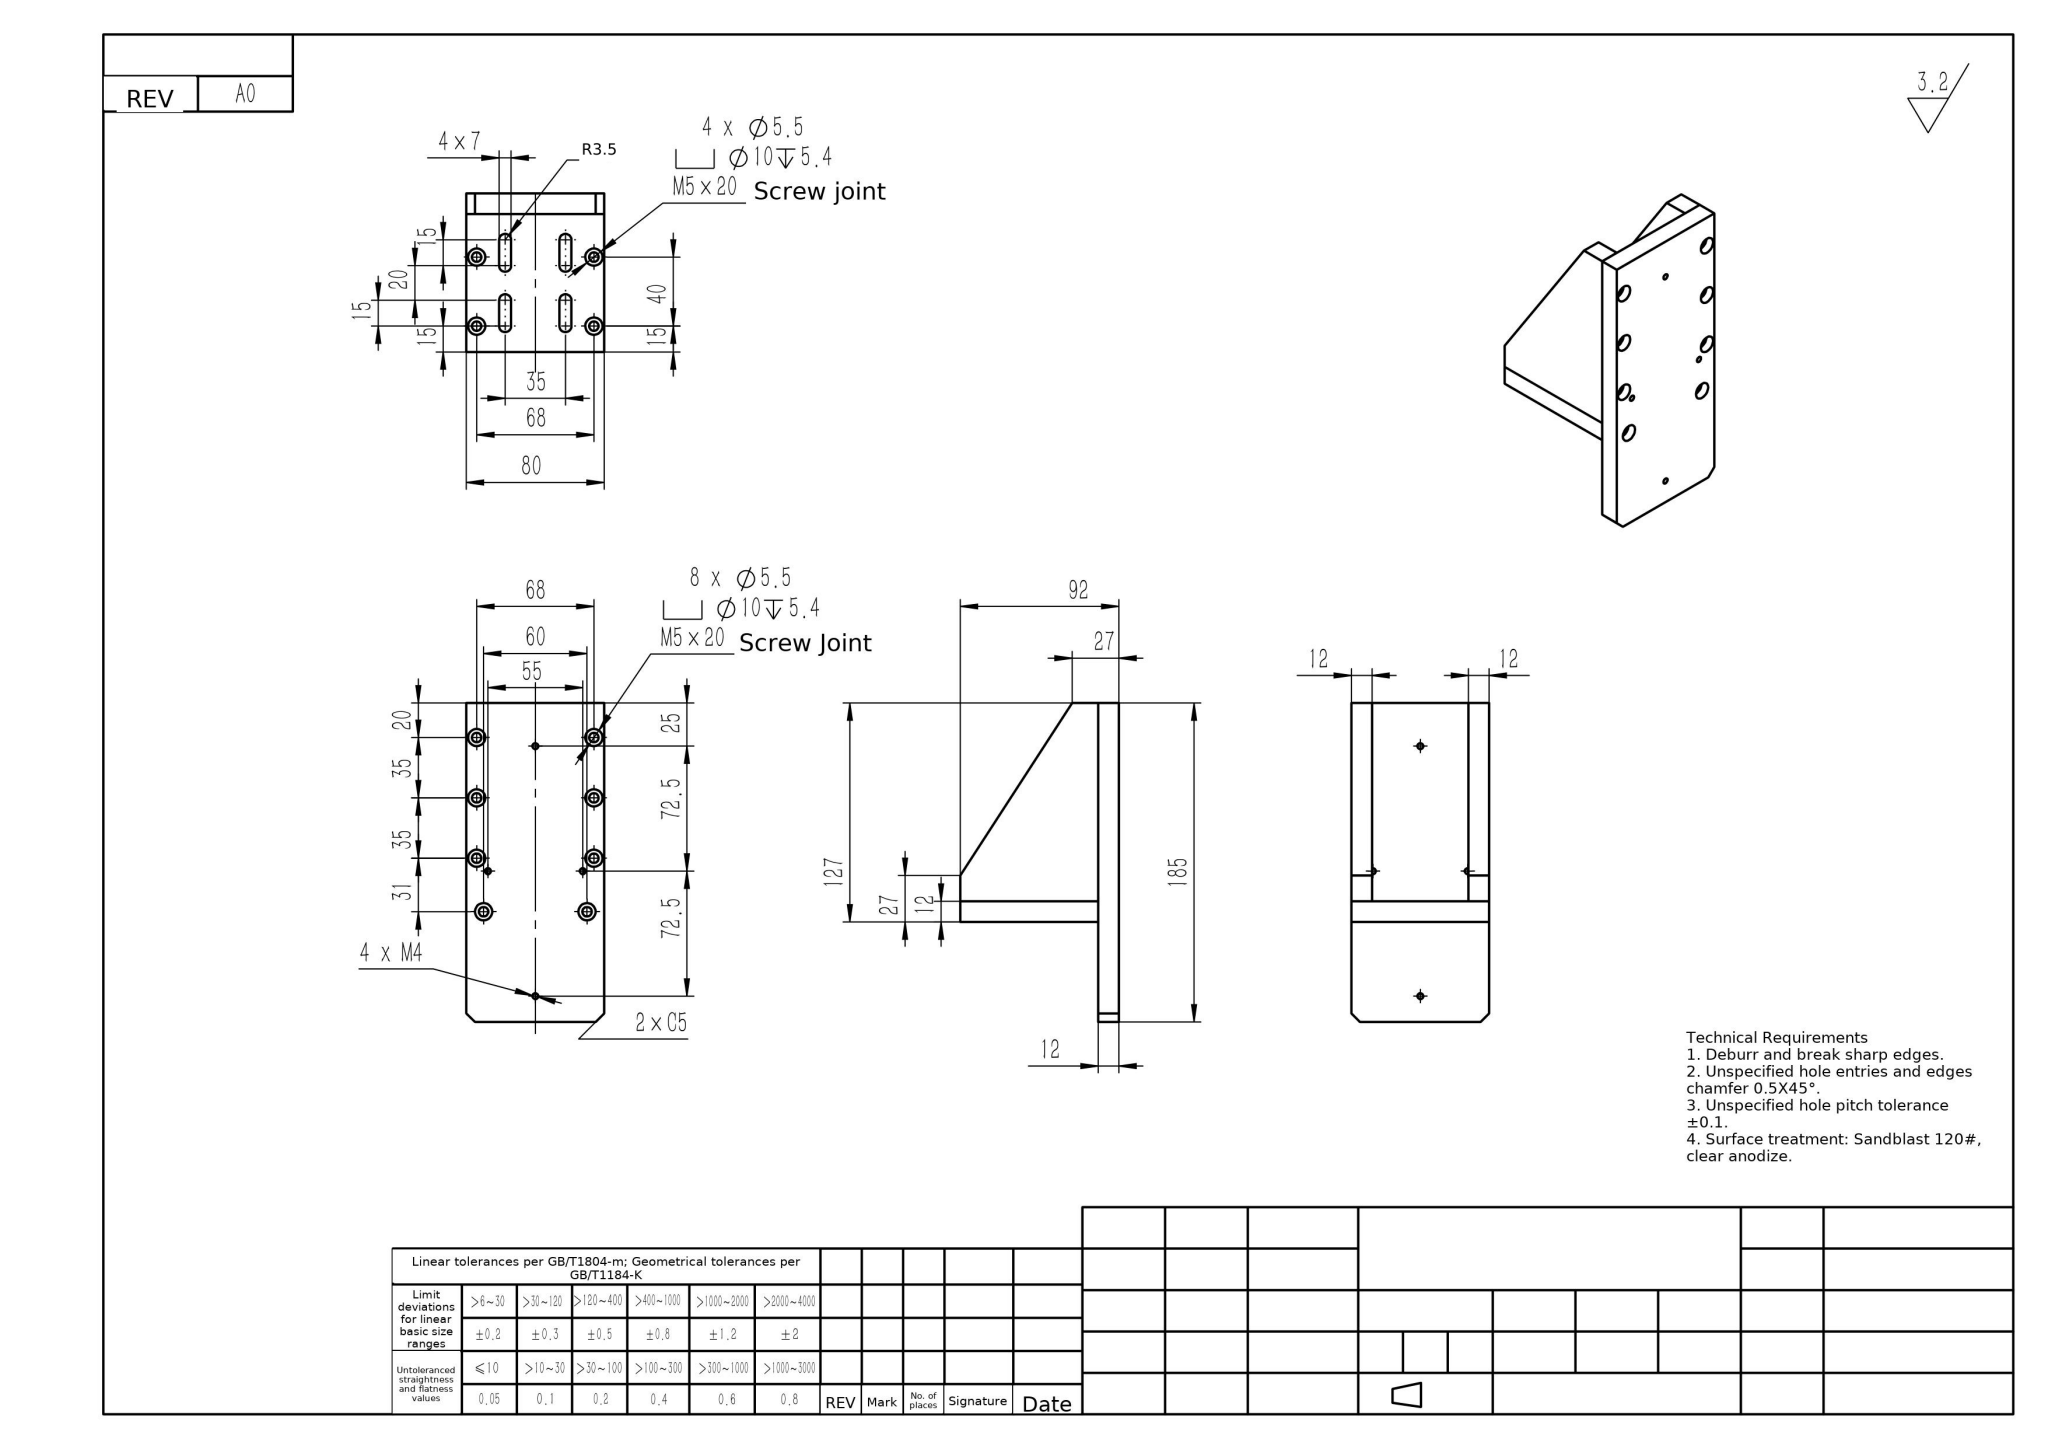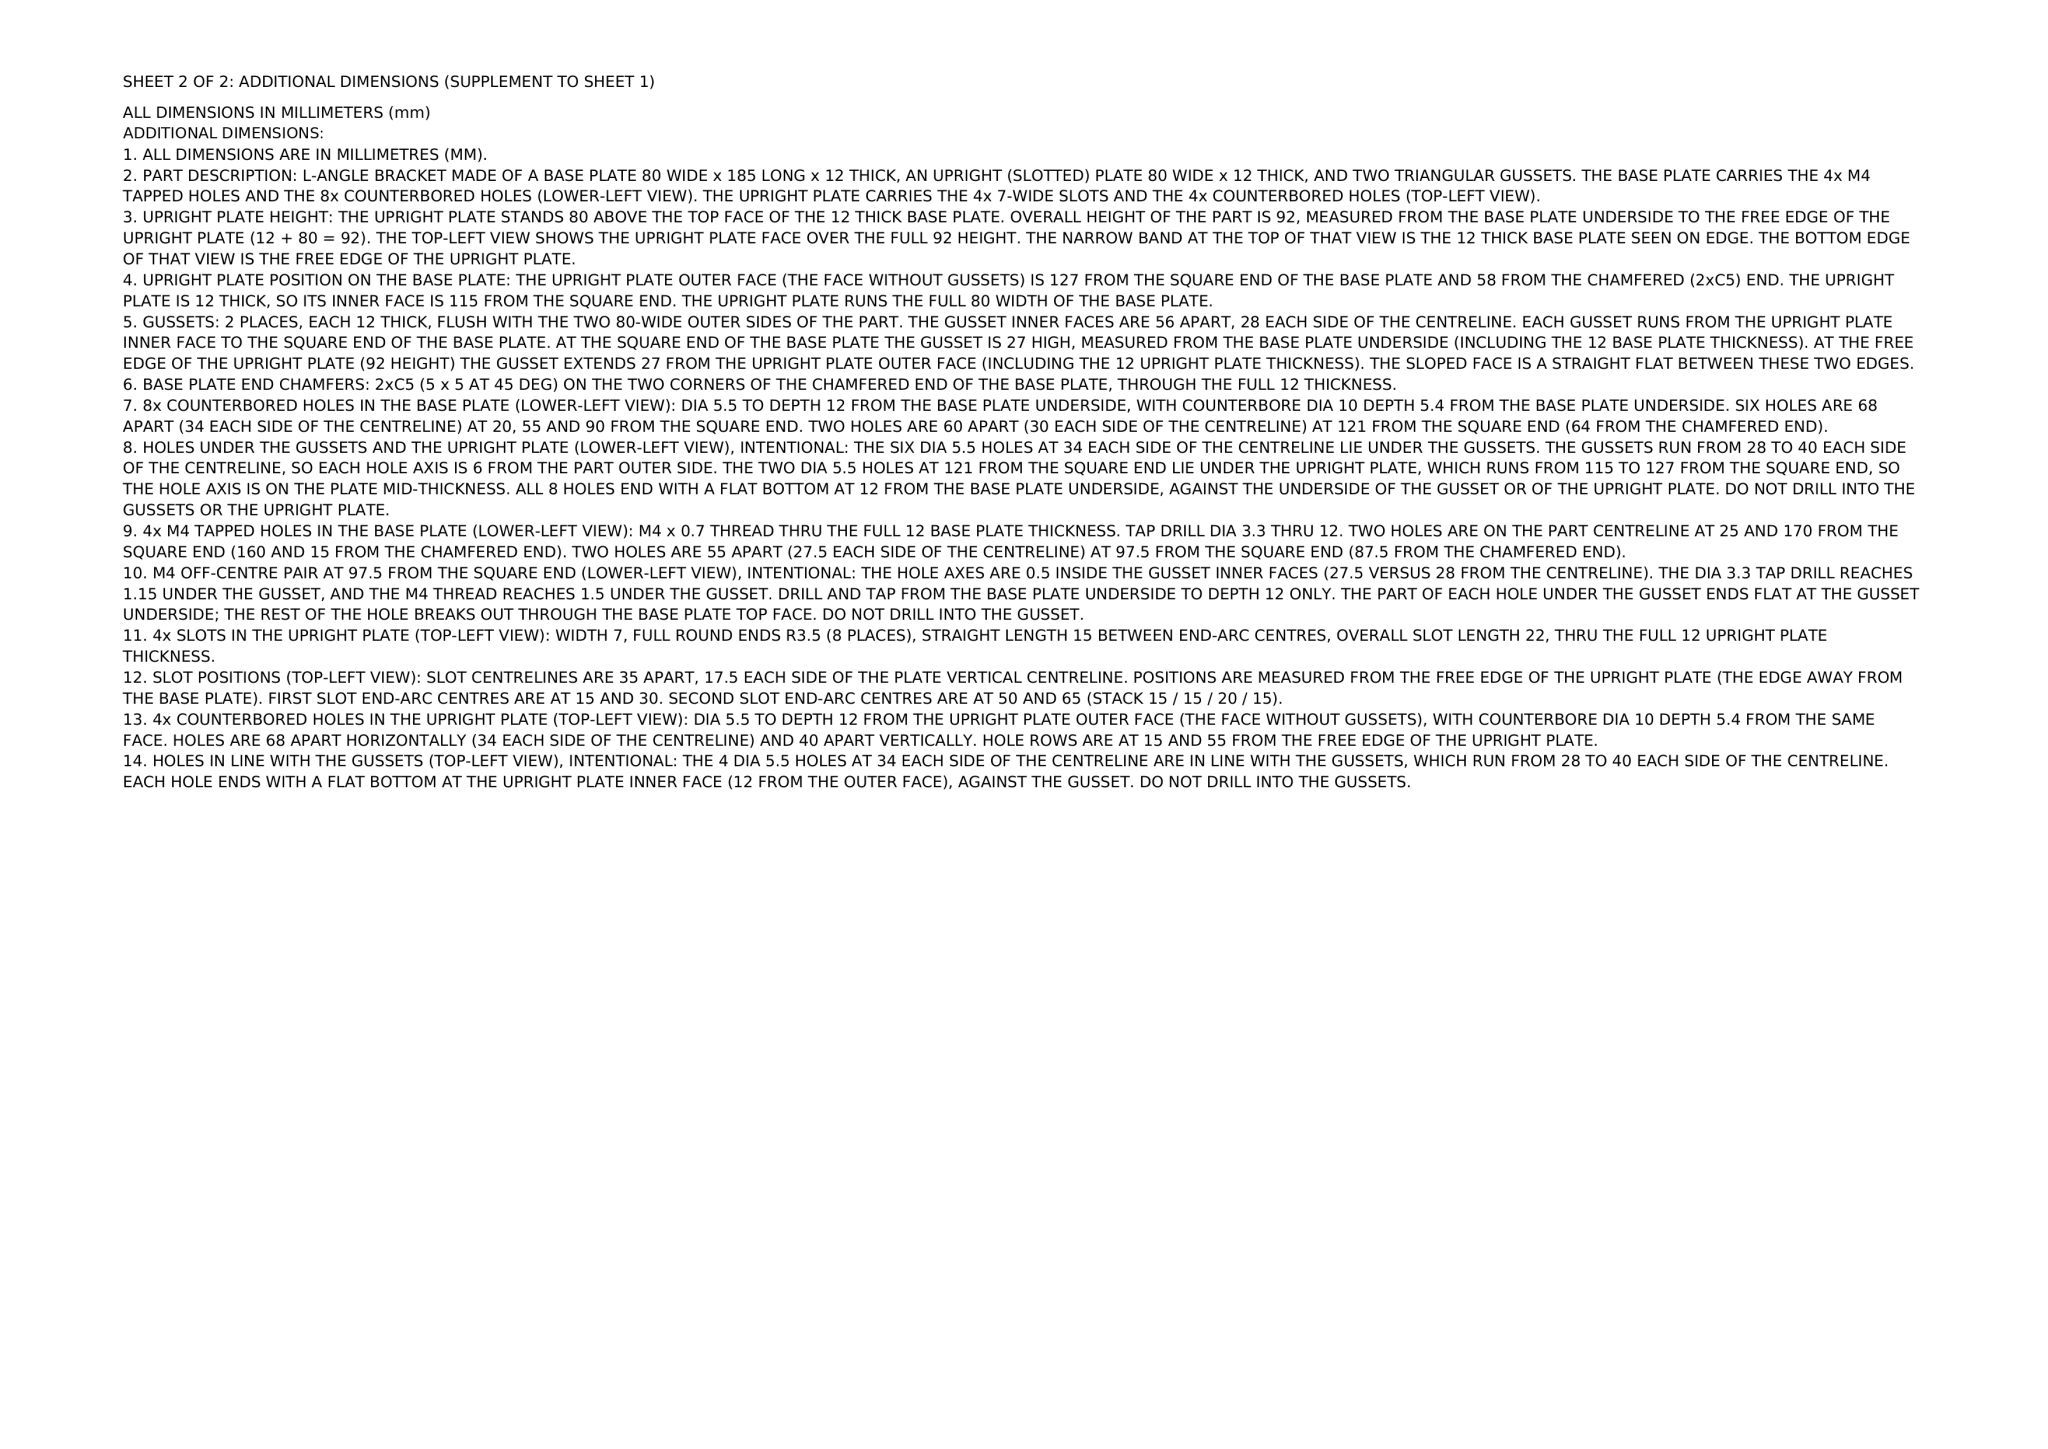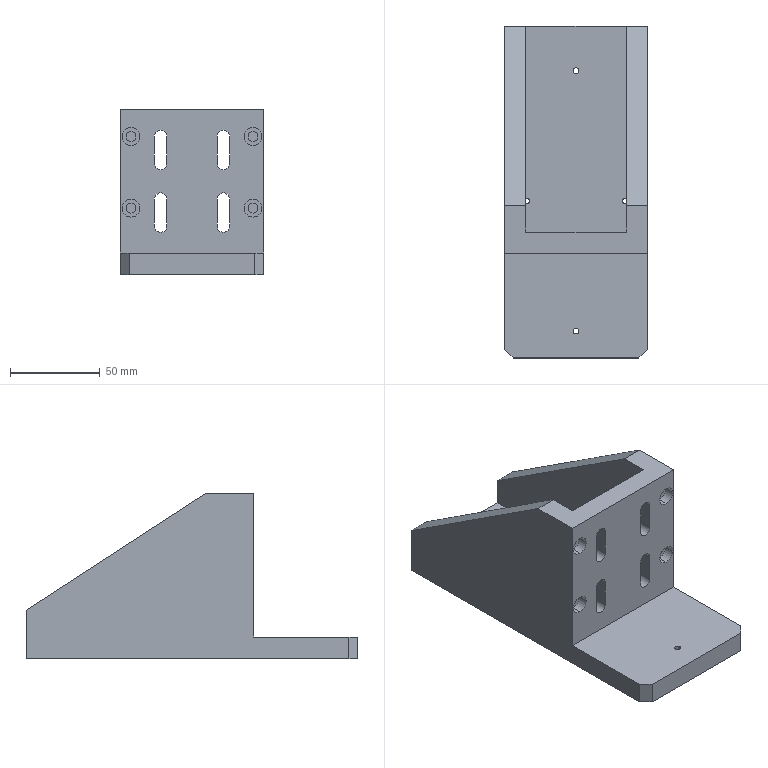Part | NX | mm | 1 solid | 114 faces | box 80 x 185 x 92 mm | volume 382631 mm3 | cylinder 64 | plane 50 | commonest cylinder face diameters 5.5 x24 10 x24 7 x8 3.3 x8